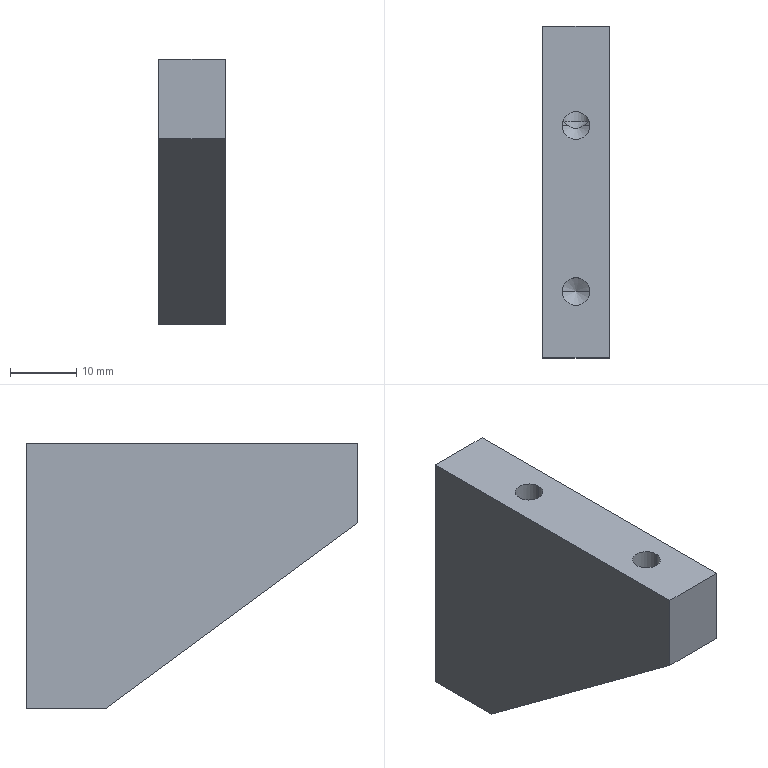Component | SolidWorks | LD101-02--Q1000-Q16-1.SLDQ1SM-1_LD101-02--Q1110-1-2 | 1 solid | 25 faces | box 10 x 50 x 40 mm | volume 13869 mm3 | cone 10 | cylinder 8 | plane 7 | commonest cylinder face diameters 4.2 x8 | material AL6061
build123d program:
from build123d import *

# Parameters (mm, degrees)
BOSS_EXTRUDE1_DEPTH   = 5
M5_TAPPED_HOLE1_D     = 4.2
M5_TAPPED_HOLE1_DEPTH = 14.4
M5_TAPPED_HOLE1_TIP   = 1.262
M5_TAPPED_HOLE2_D     = 4.2
M5_TAPPED_HOLE2_DEPTH = 14.4
M5_TAPPED_HOLE2_TIP   = 1.262


with BuildPart() as part:
    # Sketch1 → Boss-Extrude1 (new, symmetric)
    with BuildSketch(Plane.XY):
        Polygon((0, 0), (40, 0), (40, 12), (12, 50), (0, 50), align=None)
    extrude(amount=BOSS_EXTRUDE1_DEPTH, both=True)

    # M5 Tapped Hole1
    with Locations(Plane(origin=(0, 0, 0), x_dir=(-1, 0, 0), z_dir=(0, -1, 0))):
        with Locations((-15, 0), (-30, 0)):
            Hole(M5_TAPPED_HOLE1_D / 2, depth=M5_TAPPED_HOLE1_DEPTH)
            with Locations((0, 0, -(M5_TAPPED_HOLE1_DEPTH + M5_TAPPED_HOLE1_TIP / 2))):  # 118° drill point
                Cone(0, M5_TAPPED_HOLE1_D / 2, M5_TAPPED_HOLE1_TIP, mode=Mode.SUBTRACT)

    # M5 Tapped Hole2
    with Locations(Plane.ZY):
        with Locations((0, 15), (0, 40)):
            Hole(M5_TAPPED_HOLE2_D / 2, depth=M5_TAPPED_HOLE2_DEPTH)
            with Locations((0, 0, -(M5_TAPPED_HOLE2_DEPTH + M5_TAPPED_HOLE2_TIP / 2))):  # 118° drill point
                Cone(0, M5_TAPPED_HOLE2_D / 2, M5_TAPPED_HOLE2_TIP, mode=Mode.SUBTRACT)


solid = part.part

# Placed as in the assembly
solid = solid.moved(Location((-735.29, -139.897, -12.743), (180, -90, 0)))
STEP:
#1=CARTESIAN_POINT('',(-28.905,-6.098,-1.092));
#2=VERTEX_POINT('',#1);
#3=CARTESIAN_POINT('',(-28.869,-6.075,-1.069));
#4=VERTEX_POINT('',#3);
#5=CARTESIAN_POINT('',(-28.905,-6.098,-1.092));
#6=CARTESIAN_POINT('',(-28.893,-6.091,-1.085));
#7=CARTESIAN_POINT('',(-28.881,-6.083,-1.077));
#8=CARTESIAN_POINT('',(-28.869,-6.075,-1.069));
#9=B_SPLINE_CURVE_WITH_KNOTS('',3,(#5,#6,#7,#8),.UNSPECIFIED.,.F.,.F.,(4,4),(0.003787,0.005033),.UNSPECIFIED.);
#10=EDGE_CURVE('',#2,#4,#9,.T.);
#11=ORIENTED_EDGE('',*,*,#10,.F.);
#12=CARTESIAN_POINT('',(-28.866,-6.098,-1.069));
#13=VERTEX_POINT('',#12);
#14=CARTESIAN_POINT('',(-28.866,-6.098,-1.069));
#15=DIRECTION('',(0.8572,-0.,0.515));
#16=VECTOR('',#15,39.37);
#17=LINE('',#14,#16);
#18=EDGE_CURVE('',#2,#13,#17,.T.);
#19=ORIENTED_EDGE('',*,*,#18,.T.);
#20=CARTESIAN_POINT('',(-28.948,-6.098,-1.069));
#21=DIRECTION('',(-0.,-0.,1.));
#22=DIRECTION('',(-1.,0.,0.));
#23=AXIS2_PLACEMENT_3D('',#20,#21,#22);
#24=CIRCLE('',#23,0.08268);
#25=EDGE_CURVE('',#13,#4,#24,.T.);
#26=ORIENTED_EDGE('',*,*,#25,.T.);
#27=EDGE_LOOP('',(#11,#19,#26));
#28=FACE_OUTER_BOUND('',#27,.T.);
#29=CARTESIAN_POINT('',(-28.948,-6.098,-1.069));
#30=DIRECTION('',(-0.,-0.,1.));
#31=DIRECTION('',(-1.,0.,0.));
#32=AXIS2_PLACEMENT_3D('',#29,#30,#31);
#33=CONICAL_SURFACE('',#32,0.08268,1.03);
#34=ADVANCED_FACE('',(#28),#33,.F.);
#35=ORIENTED_EDGE('',*,*,#18,.F.);
#36=CARTESIAN_POINT('',(-28.992,-6.098,-1.092));
#37=VERTEX_POINT('',#36);
#38=CARTESIAN_POINT('',(-28.992,-6.098,-1.092));
#39=CARTESIAN_POINT('',(-28.985,-6.102,-1.096));
#40=CARTESIAN_POINT('',(-28.979,-6.106,-1.1));
#41=CARTESIAN_POINT('',(-28.968,-6.11,-1.104));
#42=CARTESIAN_POINT('',(-28.965,-6.112,-1.106));
#43=CARTESIAN_POINT('',(-28.957,-6.114,-1.108));
#44=CARTESIAN_POINT('',(-28.953,-6.115,-1.109));
#45=CARTESIAN_POINT('',(-28.944,-6.115,-1.109));
#46=CARTESIAN_POINT('',(-28.94,-6.114,-1.108));
#47=CARTESIAN_POINT('',(-28.932,-6.112,-1.106));
#48=CARTESIAN_POINT('',(-28.929,-6.11,-1.104));
#49=CARTESIAN_POINT('',(-28.918,-6.106,-1.1));
#50=CARTESIAN_POINT('',(-28.911,-6.102,-1.096));
#51=CARTESIAN_POINT('',(-28.905,-6.098,-1.092));
#52=B_SPLINE_CURVE_WITH_KNOTS('',3,(#38,#39,#40,#41,#42,#43,#44,#45,#46,#47,#48,#49,#50,#51),.UNSPECIFIED.,.F.,.F.,(4,2,2,2,2,2,4),(0.001245,0.001881,0.002198,0.002516,0.002834,0.003151,0.003787),.UNSPECIFIED.);
#53=EDGE_CURVE('',#37,#2,#52,.T.);
#54=ORIENTED_EDGE('',*,*,#53,.F.);
#55=CARTESIAN_POINT('',(-29.031,-6.098,-1.069));
#56=VERTEX_POINT('',#55);
#57=CARTESIAN_POINT('',(-29.031,-6.098,-1.069));
#58=DIRECTION('',(-0.8572,-0.,0.515));
#59=VECTOR('',#58,39.37);
#60=LINE('',#57,#59);
#61=EDGE_CURVE('',#37,#56,#60,.T.);
#62=ORIENTED_EDGE('',*,*,#61,.T.);
#63=CARTESIAN_POINT('',(-28.948,-6.098,-1.069));
#64=DIRECTION('',(-0.,-0.,1.));
#65=DIRECTION('',(-1.,0.,0.));
#66=AXIS2_PLACEMENT_3D('',#63,#64,#65);
#67=CIRCLE('',#66,0.08268);
#68=EDGE_CURVE('',#56,#13,#67,.T.);
#69=ORIENTED_EDGE('',*,*,#68,.T.);
#70=EDGE_LOOP('',(#35,#54,#62,#69));
#71=FACE_OUTER_BOUND('',#70,.T.);
#72=CARTESIAN_POINT('',(-28.948,-6.098,-1.069));
#73=DIRECTION('',(-0.,-0.,1.));
#74=DIRECTION('',(-1.,0.,0.));
#75=AXIS2_PLACEMENT_3D('',#72,#73,#74);
#76=CONICAL_SURFACE('',#75,0.08268,1.03);
#77=ADVANCED_FACE('',(#71),#76,.F.);
#78=ORIENTED_EDGE('',*,*,#25,.F.);
#79=CARTESIAN_POINT('',(-28.866,-6.098,-0.5017));
#80=VERTEX_POINT('',#79);
#81=CARTESIAN_POINT('',(-28.866,-6.098,-0.5017));
#82=DIRECTION('',(-0.,-0.,1.));
#83=VECTOR('',#82,39.37);
#84=LINE('',#81,#83);
#85=EDGE_CURVE('',#13,#80,#84,.T.);
#86=ORIENTED_EDGE('',*,*,#85,.T.);
#87=CARTESIAN_POINT('',(-29.031,-6.098,-0.5017));
#88=VERTEX_POINT('',#87);
#89=CARTESIAN_POINT('',(-28.948,-6.098,-0.5017));
#90=DIRECTION('',(-0.,-0.,1.));
#91=DIRECTION('',(-1.,0.,0.));
#92=AXIS2_PLACEMENT_3D('',#89,#90,#91);
#93=CIRCLE('',#92,0.08268);
#94=EDGE_CURVE('',#80,#88,#93,.T.);
#95=ORIENTED_EDGE('',*,*,#94,.T.);
#96=CARTESIAN_POINT('',(-29.031,-6.098,-0.5017));
#97=DIRECTION('',(-0.,-0.,1.));
#98=VECTOR('',#97,39.37);
#99=LINE('',#96,#98);
#100=EDGE_CURVE('',#56,#88,#99,.T.);
#101=ORIENTED_EDGE('',*,*,#100,.F.);
#102=CARTESIAN_POINT('',(-29.028,-6.075,-1.069));
#103=VERTEX_POINT('',#102);
#104=CARTESIAN_POINT('',(-28.948,-6.098,-1.069));
#105=DIRECTION('',(-0.,-0.,1.));
#106=DIRECTION('',(-1.,0.,0.));
#107=AXIS2_PLACEMENT_3D('',#104,#105,#106);
#108=CIRCLE('',#107,0.08268);
#109=EDGE_CURVE('',#103,#56,#108,.T.);
#110=ORIENTED_EDGE('',*,*,#109,.F.);
#111=CARTESIAN_POINT('',(-28.869,-6.075,-1.069));
#112=CARTESIAN_POINT('',(-28.898,-5.978,-0.972));
#113=CARTESIAN_POINT('',(-28.999,-5.978,-0.972));
#114=CARTESIAN_POINT('',(-29.028,-6.075,-1.069));
#115=(BOUNDED_CURVE()B_SPLINE_CURVE(3,(#111,#112,#113,#114),.UNSPECIFIED.,.F.,.T.)B_SPLINE_CURVE_WITH_KNOTS((4,4),(5.002,7.564),.UNSPECIFIED.)CURVE()GEOMETRIC_REPRESENTATION_ITEM()RATIONAL_B_SPLINE_CURVE((1.,0.5238,0.5238,1.))REPRESENTATION_ITEM(''));
#116=EDGE_CURVE('',#4,#103,#115,.T.);
#117=ORIENTED_EDGE('',*,*,#116,.F.);
#118=EDGE_LOOP('',(#78,#86,#95,#101,#110,#117));
#119=FACE_OUTER_BOUND('',#118,.T.);
#120=CARTESIAN_POINT('',(-28.948,-6.098,-0.5017));
#121=DIRECTION('',(-0.,-0.,1.));
#122=DIRECTION('',(-1.,0.,0.));
#123=AXIS2_PLACEMENT_3D('',#120,#121,#122);
#124=CYLINDRICAL_SURFACE('',#123,0.08268);
#125=ADVANCED_FACE('',(#119),#124,.F.);
#126=CARTESIAN_POINT('',(-28.866,-7.083,-1.069));
#127=VERTEX_POINT('',#126);
#128=CARTESIAN_POINT('',(-29.031,-7.083,-1.069));
#129=VERTEX_POINT('',#128);
#130=CARTESIAN_POINT('',(-28.948,-7.083,-1.069));
#131=DIRECTION('',(-0.,-0.,1.));
#132=DIRECTION('',(-1.,0.,0.));
#133=AXIS2_PLACEMENT_3D('',#130,#131,#132);
#134=CIRCLE('',#133,0.08268);
#135=EDGE_CURVE('',#127,#129,#134,.T.);
#136=ORIENTED_EDGE('',*,*,#135,.F.);
#137=CARTESIAN_POINT('',(-28.866,-7.083,-0.5017));
#138=VERTEX_POINT('',#137);
#139=CARTESIAN_POINT('',(-28.866,-7.083,-0.5017));
#140=DIRECTION('',(-0.,-0.,1.));
#141=VECTOR('',#140,39.37);
#142=LINE('',#139,#141);
#143=EDGE_CURVE('',#127,#138,#142,.T.);
#144=ORIENTED_EDGE('',*,*,#143,.T.);
#145=CARTESIAN_POINT('',(-29.031,-7.083,-0.5017));
#146=VERTEX_POINT('',#145);
#147=CARTESIAN_POINT('',(-28.948,-7.083,-0.5017));
#148=DIRECTION('',(-0.,-0.,1.));
#149=DIRECTION('',(-1.,0.,0.));
#150=AXIS2_PLACEMENT_3D('',#147,#148,#149);
#151=CIRCLE('',#150,0.08268);
#152=EDGE_CURVE('',#138,#146,#151,.T.);
#153=ORIENTED_EDGE('',*,*,#152,.T.);
#154=CARTESIAN_POINT('',(-29.031,-7.083,-0.5017));
#155=DIRECTION('',(-0.,-0.,1.));
#156=VECTOR('',#155,39.37);
#157=LINE('',#154,#156);
#158=EDGE_CURVE('',#129,#146,#157,.T.);
#159=ORIENTED_EDGE('',*,*,#158,.F.);
#160=EDGE_LOOP('',(#136,#144,#153,#159));
#161=FACE_OUTER_BOUND('',#160,.T.);
#162=CARTESIAN_POINT('',(-28.948,-7.083,-0.5017));
#163=DIRECTION('',(-0.,-0.,1.));
#164=DIRECTION('',(-1.,0.,0.));
#165=AXIS2_PLACEMENT_3D('',#162,#163,#164);
#166=CYLINDRICAL_SURFACE('',#165,0.08268);
#167=ADVANCED_FACE('',(#161),#166,.F.);
#168=CARTESIAN_POINT('',(-28.948,-7.083,-1.118));
#169=VERTEX_POINT('',#168);
#170=CARTESIAN_POINT('',(-29.031,-7.083,-1.069));
#171=DIRECTION('',(-0.8572,-0.,0.515));
#172=VECTOR('',#171,39.37);
#173=LINE('',#170,#172);
#174=EDGE_CURVE('',#169,#129,#173,.T.);
#175=ORIENTED_EDGE('',*,*,#174,.F.);
#176=CARTESIAN_POINT('',(-28.866,-7.083,-1.069));
#177=DIRECTION('',(0.8572,-0.,0.515));
#178=VECTOR('',#177,39.37);
#179=LINE('',#176,#178);
#180=EDGE_CURVE('',#169,#127,#179,.T.);
#181=ORIENTED_EDGE('',*,*,#180,.T.);
#182=ORIENTED_EDGE('',*,*,#135,.T.);
#183=EDGE_LOOP('',(#175,#181,#182));
#184=FACE_OUTER_BOUND('',#183,.T.);
#185=CARTESIAN_POINT('',(-28.948,-7.083,-1.069));
#186=DIRECTION('',(-0.,-0.,1.));
#187=DIRECTION('',(-1.,0.,0.));
#188=AXIS2_PLACEMENT_3D('',#185,#186,#187);
#189=CONICAL_SURFACE('',#188,0.08268,1.03);
#190=ADVANCED_FACE('',(#184),#189,.F.);
#191=CARTESIAN_POINT('',(-29.031,-6.075,-1.092));
#192=VERTEX_POINT('',#191);
#193=CARTESIAN_POINT('',(-28.948,-6.075,-1.092));
#194=DIRECTION('',(0.,1.,0.));
#195=DIRECTION('',(1.,0.,0.));
#196=AXIS2_PLACEMENT_3D('',#193,#194,#195);
#197=CIRCLE('',#196,0.08268);
#198=EDGE_CURVE('',#192,#103,#197,.T.);
#199=ORIENTED_EDGE('',*,*,#198,.F.);
#200=CARTESIAN_POINT('',(-29.031,-5.508,-1.092));
#201=VERTEX_POINT('',#200);
#202=CARTESIAN_POINT('',(-29.031,-5.508,-1.092));
#203=DIRECTION('',(0.,1.,0.));
#204=VECTOR('',#203,39.37);
#205=LINE('',#202,#204);
#206=EDGE_CURVE('',#192,#201,#205,.T.);
#207=ORIENTED_EDGE('',*,*,#206,.T.);
#208=CARTESIAN_POINT('',(-28.866,-5.508,-1.092));
#209=VERTEX_POINT('',#208);
#210=CARTESIAN_POINT('',(-28.948,-5.508,-1.092));
#211=DIRECTION('',(0.,1.,0.));
#212=DIRECTION('',(1.,0.,0.));
#213=AXIS2_PLACEMENT_3D('',#210,#211,#212);
#214=CIRCLE('',#213,0.08268);
#215=EDGE_CURVE('',#201,#209,#214,.T.);
#216=ORIENTED_EDGE('',*,*,#215,.T.);
#217=CARTESIAN_POINT('',(-28.866,-6.075,-1.092));
#218=VERTEX_POINT('',#217);
#219=CARTESIAN_POINT('',(-28.866,-5.508,-1.092));
#220=DIRECTION('',(0.,1.,0.));
#221=VECTOR('',#220,39.37);
#222=LINE('',#219,#221);
#223=EDGE_CURVE('',#218,#209,#222,.T.);
#224=ORIENTED_EDGE('',*,*,#223,.F.);
#225=CARTESIAN_POINT('',(-28.948,-6.075,-1.092));
#226=DIRECTION('',(0.,1.,0.));
#227=DIRECTION('',(1.,0.,0.));
#228=AXIS2_PLACEMENT_3D('',#225,#226,#227);
#229=CIRCLE('',#228,0.08268);
#230=EDGE_CURVE('',#4,#218,#229,.T.);
#231=ORIENTED_EDGE('',*,*,#230,.F.);
#232=ORIENTED_EDGE('',*,*,#116,.T.);
#233=EDGE_LOOP('',(#199,#207,#216,#224,#231,#232));
#234=FACE_OUTER_BOUND('',#233,.T.);
#235=CARTESIAN_POINT('',(-28.948,-5.508,-1.092));
#236=DIRECTION('',(0.,1.,0.));
#237=DIRECTION('',(1.,0.,0.));
#238=AXIS2_PLACEMENT_3D('',#235,#236,#237);
#239=CYLINDRICAL_SURFACE('',#238,0.08268);
#240=ADVANCED_FACE('',(#234),#239,.F.);
#241=CARTESIAN_POINT('',(-29.028,-6.075,-1.069));
#242=CARTESIAN_POINT('',(-29.016,-6.083,-1.077));
#243=CARTESIAN_POINT('',(-29.004,-6.091,-1.085));
#244=CARTESIAN_POINT('',(-28.992,-6.098,-1.092));
#245=B_SPLINE_CURVE_WITH_KNOTS('',3,(#241,#242,#243,#244),.UNSPECIFIED.,.F.,.F.,(4,4),(0.0000004,0.001245),.UNSPECIFIED.);
#246=EDGE_CURVE('',#103,#37,#245,.T.);
#247=ORIENTED_EDGE('',*,*,#246,.T.);
#248=CARTESIAN_POINT('',(-29.031,-6.075,-1.092));
#249=DIRECTION('',(-0.8572,0.515,-0.));
#250=VECTOR('',#249,39.37);
#251=LINE('',#248,#250);
#252=EDGE_CURVE('',#37,#192,#251,.T.);
#253=ORIENTED_EDGE('',*,*,#252,.T.);
#254=ORIENTED_EDGE('',*,*,#198,.T.);
#255=EDGE_LOOP('',(#247,#253,#254));
#256=FACE_OUTER_BOUND('',#255,.T.);
#257=CARTESIAN_POINT('',(-28.948,-6.075,-1.092));
#258=DIRECTION('',(0.,1.,0.));
#259=DIRECTION('',(1.,0.,0.));
#260=AXIS2_PLACEMENT_3D('',#257,#258,#259);
#261=CONICAL_SURFACE('',#260,0.08268,1.03);
#262=ADVANCED_FACE('',(#256),#261,.F.);
#263=ORIENTED_EDGE('',*,*,#252,.F.);
#264=ORIENTED_EDGE('',*,*,#53,.T.);
#265=CARTESIAN_POINT('',(-28.866,-6.075,-1.092));
#266=DIRECTION('',(0.8572,0.515,0.));
#267=VECTOR('',#266,39.37);
#268=LINE('',#265,#267);
#269=EDGE_CURVE('',#2,#218,#268,.T.);
#270=ORIENTED_EDGE('',*,*,#269,.T.);
#271=CARTESIAN_POINT('',(-28.948,-6.075,-1.092));
#272=DIRECTION('',(0.,1.,0.));
#273=DIRECTION('',(1.,0.,0.));
#274=AXIS2_PLACEMENT_3D('',#271,#272,#273);
#275=CIRCLE('',#274,0.08268);
#276=EDGE_CURVE('',#218,#192,#275,.T.);
#277=ORIENTED_EDGE('',*,*,#276,.T.);
#278=EDGE_LOOP('',(#263,#264,#270,#277));
#279=FACE_OUTER_BOUND('',#278,.T.);
#280=CARTESIAN_POINT('',(-28.948,-6.075,-1.092));
#281=DIRECTION('',(0.,1.,0.));
#282=DIRECTION('',(1.,0.,0.));
#283=AXIS2_PLACEMENT_3D('',#280,#281,#282);
#284=CONICAL_SURFACE('',#283,0.08268,1.03);
#285=ADVANCED_FACE('',(#279),#284,.F.);
#286=CARTESIAN_POINT('',(-29.031,-6.075,-1.683));
#287=VERTEX_POINT('',#286);
#288=CARTESIAN_POINT('',(-28.866,-6.075,-1.683));
#289=VERTEX_POINT('',#288);
#290=CARTESIAN_POINT('',(-28.948,-6.075,-1.683));
#291=DIRECTION('',(0.,1.,0.));
#292=DIRECTION('',(1.,0.,0.));
#293=AXIS2_PLACEMENT_3D('',#290,#291,#292);
#294=CIRCLE('',#293,0.08268);
#295=EDGE_CURVE('',#287,#289,#294,.T.);
#296=ORIENTED_EDGE('',*,*,#295,.F.);
#297=CARTESIAN_POINT('',(-29.031,-5.508,-1.683));
#298=VERTEX_POINT('',#297);
#299=CARTESIAN_POINT('',(-29.031,-5.508,-1.683));
#300=DIRECTION('',(0.,1.,0.));
#301=VECTOR('',#300,39.37);
#302=LINE('',#299,#301);
#303=EDGE_CURVE('',#287,#298,#302,.T.);
#304=ORIENTED_EDGE('',*,*,#303,.T.);
#305=CARTESIAN_POINT('',(-28.866,-5.508,-1.683));
#306=VERTEX_POINT('',#305);
#307=CARTESIAN_POINT('',(-28.948,-5.508,-1.683));
#308=DIRECTION('',(0.,1.,0.));
#309=DIRECTION('',(1.,0.,0.));
#310=AXIS2_PLACEMENT_3D('',#307,#308,#309);
#311=CIRCLE('',#310,0.08268);
#312=EDGE_CURVE('',#298,#306,#311,.T.);
#313=ORIENTED_EDGE('',*,*,#312,.T.);
#314=CARTESIAN_POINT('',(-28.866,-5.508,-1.683));
#315=DIRECTION('',(0.,1.,0.));
#316=VECTOR('',#315,39.37);
#317=LINE('',#314,#316);
#318=EDGE_CURVE('',#289,#306,#317,.T.);
#319=ORIENTED_EDGE('',*,*,#318,.F.);
#320=EDGE_LOOP('',(#296,#304,#313,#319));
#321=FACE_OUTER_BOUND('',#320,.T.);
#322=CARTESIAN_POINT('',(-28.948,-5.508,-1.683));
#323=DIRECTION('',(0.,1.,0.));
#324=DIRECTION('',(1.,0.,0.));
#325=AXIS2_PLACEMENT_3D('',#322,#323,#324);
#326=CYLINDRICAL_SURFACE('',#325,0.08268);
#327=ADVANCED_FACE('',(#321),#326,.F.);
#328=CARTESIAN_POINT('',(-28.948,-6.124,-1.683));
#329=VERTEX_POINT('',#328);
#330=CARTESIAN_POINT('',(-28.866,-6.075,-1.683));
#331=DIRECTION('',(0.8572,0.515,0.));
#332=VECTOR('',#331,39.37);
#333=LINE('',#330,#332);
#334=EDGE_CURVE('',#329,#289,#333,.T.);
#335=ORIENTED_EDGE('',*,*,#334,.F.);
#336=CARTESIAN_POINT('',(-29.031,-6.075,-1.683));
#337=DIRECTION('',(-0.8572,0.515,-0.));
#338=VECTOR('',#337,39.37);
#339=LINE('',#336,#338);
#340=EDGE_CURVE('',#329,#287,#339,.T.);
#341=ORIENTED_EDGE('',*,*,#340,.T.);
#342=ORIENTED_EDGE('',*,*,#295,.T.);
#343=EDGE_LOOP('',(#335,#341,#342));
#344=FACE_OUTER_BOUND('',#343,.T.);
#345=CARTESIAN_POINT('',(-28.948,-6.075,-1.683));
#346=DIRECTION('',(0.,1.,0.));
#347=DIRECTION('',(1.,0.,0.));
#348=AXIS2_PLACEMENT_3D('',#345,#346,#347);
#349=CONICAL_SURFACE('',#348,0.08268,1.03);
#350=ADVANCED_FACE('',(#344),#349,.F.);
#351=CARTESIAN_POINT('',(-28.948,-6.098,-0.5017));
#352=DIRECTION('',(-0.,-0.,1.));
#353=DIRECTION('',(-1.,0.,0.));
#354=AXIS2_PLACEMENT_3D('',#351,#352,#353);
#355=CIRCLE('',#354,0.08268);
#356=EDGE_CURVE('',#88,#80,#355,.T.);
#357=ORIENTED_EDGE('',*,*,#356,.F.);
#358=ORIENTED_EDGE('',*,*,#94,.F.);
#359=EDGE_LOOP('',(#357,#358));
#360=FACE_BOUND('',#359,.T.);
#361=CARTESIAN_POINT('',(-28.948,-7.083,-0.5017));
#362=DIRECTION('',(-0.,-0.,1.));
#363=DIRECTION('',(-1.,0.,0.));
#364=AXIS2_PLACEMENT_3D('',#361,#362,#363);
#365=CIRCLE('',#364,0.08268);
#366=EDGE_CURVE('',#146,#138,#365,.T.);
#367=ORIENTED_EDGE('',*,*,#366,.F.);
#368=ORIENTED_EDGE('',*,*,#152,.F.);
#369=EDGE_LOOP('',(#367,#368));
#370=FACE_BOUND('',#369,.T.);
#371=CARTESIAN_POINT('',(-28.752,-7.476,-0.5017));
#372=VERTEX_POINT('',#371);
#373=CARTESIAN_POINT('',(-28.752,-5.508,-0.5017));
#374=VERTEX_POINT('',#373);
#375=CARTESIAN_POINT('',(-28.752,-7.476,-0.5017));
#376=DIRECTION('',(0.,1.,-0.));
#377=VECTOR('',#376,39.37);
#378=LINE('',#375,#377);
#379=EDGE_CURVE('',#372,#374,#378,.T.);
#380=ORIENTED_EDGE('',*,*,#379,.T.);
#381=CARTESIAN_POINT('',(-29.145,-5.508,-0.5017));
#382=VERTEX_POINT('',#381);
#383=CARTESIAN_POINT('',(-29.145,-5.508,-0.5017));
#384=DIRECTION('',(1.,-0.,0.));
#385=VECTOR('',#384,39.37);
#386=LINE('',#383,#385);
#387=EDGE_CURVE('',#382,#374,#386,.T.);
#388=ORIENTED_EDGE('',*,*,#387,.F.);
#389=CARTESIAN_POINT('',(-29.145,-7.476,-0.5017));
#390=VERTEX_POINT('',#389);
#391=CARTESIAN_POINT('',(-29.145,-7.476,-0.5017));
#392=DIRECTION('',(0.,1.,-0.));
#393=VECTOR('',#392,39.37);
#394=LINE('',#391,#393);
#395=EDGE_CURVE('',#390,#382,#394,.T.);
#396=ORIENTED_EDGE('',*,*,#395,.F.);
#397=CARTESIAN_POINT('',(-29.145,-7.476,-0.5017));
#398=DIRECTION('',(1.,-0.,0.));
#399=VECTOR('',#398,39.37);
#400=LINE('',#397,#399);
#401=EDGE_CURVE('',#390,#372,#400,.T.);
#402=ORIENTED_EDGE('',*,*,#401,.T.);
#403=EDGE_LOOP('',(#380,#388,#396,#402));
#404=FACE_OUTER_BOUND('',#403,.T.);
#405=CARTESIAN_POINT('',(-29.145,-7.476,-0.5017));
#406=DIRECTION('',(0.,-0.,-1.));
#407=DIRECTION('',(-0.,-1.,0.));
#408=AXIS2_PLACEMENT_3D('',#405,#406,#407);
#409=PLANE('',#408);
#410=ADVANCED_FACE('',(#360,#370,#404),#409,.F.);
#411=CARTESIAN_POINT('',(-28.948,-5.508,-1.092));
#412=DIRECTION('',(0.,1.,0.));
#413=DIRECTION('',(1.,0.,0.));
#414=AXIS2_PLACEMENT_3D('',#411,#412,#413);
#415=CIRCLE('',#414,0.08268);
#416=EDGE_CURVE('',#209,#201,#415,.T.);
#417=ORIENTED_EDGE('',*,*,#416,.F.);
#418=ORIENTED_EDGE('',*,*,#215,.F.);
#419=EDGE_LOOP('',(#417,#418));
#420=FACE_BOUND('',#419,.T.);
#421=CARTESIAN_POINT('',(-28.948,-5.508,-1.683));
#422=DIRECTION('',(0.,1.,0.));
#423=DIRECTION('',(1.,0.,0.));
#424=AXIS2_PLACEMENT_3D('',#421,#422,#423);
#425=CIRCLE('',#424,0.08268);
#426=EDGE_CURVE('',#306,#298,#425,.T.);
#427=ORIENTED_EDGE('',*,*,#426,.F.);
#428=ORIENTED_EDGE('',*,*,#312,.F.);
#429=EDGE_LOOP('',(#427,#428));
#430=FACE_BOUND('',#429,.T.);
#431=CARTESIAN_POINT('',(-28.752,-5.508,-2.077));
#432=VERTEX_POINT('',#431);
#433=CARTESIAN_POINT('',(-28.752,-5.508,-0.5017));
#434=DIRECTION('',(0.,0.,-1.));
#435=VECTOR('',#434,39.37);
#436=LINE('',#433,#435);
#437=EDGE_CURVE('',#374,#432,#436,.T.);
#438=ORIENTED_EDGE('',*,*,#437,.T.);
#439=CARTESIAN_POINT('',(-29.145,-5.508,-2.077));
#440=VERTEX_POINT('',#439);
#441=CARTESIAN_POINT('',(-29.145,-5.508,-2.077));
#442=DIRECTION('',(1.,-0.,0.));
#443=VECTOR('',#442,39.37);
#444=LINE('',#441,#443);
#445=EDGE_CURVE('',#440,#432,#444,.T.);
#446=ORIENTED_EDGE('',*,*,#445,.F.);
#447=CARTESIAN_POINT('',(-29.145,-5.508,-0.5017));
#448=DIRECTION('',(0.,0.,-1.));
#449=VECTOR('',#448,39.37);
#450=LINE('',#447,#449);
#451=EDGE_CURVE('',#382,#440,#450,.T.);
#452=ORIENTED_EDGE('',*,*,#451,.F.);
#453=ORIENTED_EDGE('',*,*,#387,.T.);
#454=EDGE_LOOP('',(#438,#446,#452,#453));
#455=FACE_OUTER_BOUND('',#454,.T.);
#456=CARTESIAN_POINT('',(-29.145,-5.508,-0.5017));
#457=DIRECTION('',(-0.,-1.,-0.));
#458=DIRECTION('',(-1.,0.,-0.));
#459=AXIS2_PLACEMENT_3D('',#456,#457,#458);
#460=PLANE('',#459);
#461=ADVANCED_FACE('',(#420,#430,#455),#460,.F.);
#462=CARTESIAN_POINT('',(-28.752,-5.98,-2.077));
#463=VERTEX_POINT('',#462);
#464=CARTESIAN_POINT('',(-28.752,-5.508,-2.077));
#465=DIRECTION('',(-0.,-1.,-0.));
#466=VECTOR('',#465,39.37);
#467=LINE('',#464,#466);
#468=EDGE_CURVE('',#432,#463,#467,.T.);
#469=ORIENTED_EDGE('',*,*,#468,.T.);
#470=CARTESIAN_POINT('',(-29.145,-5.98,-2.077));
#471=VERTEX_POINT('',#470);
#472=CARTESIAN_POINT('',(-29.145,-5.98,-2.077));
#473=DIRECTION('',(1.,-0.,0.));
#474=VECTOR('',#473,39.37);
#475=LINE('',#472,#474);
#476=EDGE_CURVE('',#471,#463,#475,.T.);
#477=ORIENTED_EDGE('',*,*,#476,.F.);
#478=CARTESIAN_POINT('',(-29.145,-5.508,-2.077));
#479=DIRECTION('',(-0.,-1.,-0.));
#480=VECTOR('',#479,39.37);
#481=LINE('',#478,#480);
#482=EDGE_CURVE('',#440,#471,#481,.T.);
#483=ORIENTED_EDGE('',*,*,#482,.F.);
#484=ORIENTED_EDGE('',*,*,#445,.T.);
#485=EDGE_LOOP('',(#469,#477,#483,#484));
#486=FACE_OUTER_BOUND('',#485,.T.);
#487=CARTESIAN_POINT('',(-29.145,-5.508,-2.077));
#488=DIRECTION('',(-0.,-0.,1.));
#489=DIRECTION('',(-1.,0.,-0.));
#490=AXIS2_PLACEMENT_3D('',#487,#488,#489);
#491=PLANE('',#490);
#492=ADVANCED_FACE('',(#486),#491,.F.);
#493=CARTESIAN_POINT('',(-28.752,-7.476,-0.9741));
#494=VERTEX_POINT('',#493);
#495=CARTESIAN_POINT('',(-28.752,-5.98,-2.077));
#496=DIRECTION('',(-0.,-0.8051,0.5932));
#497=VECTOR('',#496,39.37);
#498=LINE('',#495,#497);
#499=EDGE_CURVE('',#463,#494,#498,.T.);
#500=ORIENTED_EDGE('',*,*,#499,.T.);
#501=CARTESIAN_POINT('',(-29.145,-7.476,-0.9741));
#502=VERTEX_POINT('',#501);
#503=CARTESIAN_POINT('',(-29.145,-7.476,-0.9741));
#504=DIRECTION('',(1.,-0.,0.));
#505=VECTOR('',#504,39.37);
#506=LINE('',#503,#505);
#507=EDGE_CURVE('',#502,#494,#506,.T.);
#508=ORIENTED_EDGE('',*,*,#507,.F.);
#509=CARTESIAN_POINT('',(-29.145,-5.98,-2.077));
#510=DIRECTION('',(-0.,-0.8051,0.5932));
#511=VECTOR('',#510,39.37);
#512=LINE('',#509,#511);
#513=EDGE_CURVE('',#471,#502,#512,.T.);
#514=ORIENTED_EDGE('',*,*,#513,.F.);
#515=ORIENTED_EDGE('',*,*,#476,.T.);
#516=EDGE_LOOP('',(#500,#508,#514,#515));
#517=FACE_OUTER_BOUND('',#516,.T.);
#518=CARTESIAN_POINT('',(-29.145,-5.98,-2.077));
#519=DIRECTION('',(-0.,0.5932,0.8051));
#520=DIRECTION('',(0.,0.8051,-0.5932));
#521=AXIS2_PLACEMENT_3D('',#518,#519,#520);
#522=PLANE('',#521);
#523=ADVANCED_FACE('',(#517),#522,.F.);
#524=CARTESIAN_POINT('',(-28.752,-7.476,-0.9741));
#525=DIRECTION('',(-0.,-0.,1.));
#526=VECTOR('',#525,39.37);
#527=LINE('',#524,#526);
#528=EDGE_CURVE('',#494,#372,#527,.T.);
#529=ORIENTED_EDGE('',*,*,#528,.T.);
#530=ORIENTED_EDGE('',*,*,#401,.F.);
#531=CARTESIAN_POINT('',(-29.145,-7.476,-0.9741));
#532=DIRECTION('',(-0.,-0.,1.));
#533=VECTOR('',#532,39.37);
#534=LINE('',#531,#533);
#535=EDGE_CURVE('',#502,#390,#534,.T.);
#536=ORIENTED_EDGE('',*,*,#535,.F.);
#537=ORIENTED_EDGE('',*,*,#507,.T.);
#538=EDGE_LOOP('',(#529,#530,#536,#537));
#539=FACE_OUTER_BOUND('',#538,.T.);
#540=CARTESIAN_POINT('',(-29.145,-7.476,-0.9741));
#541=DIRECTION('',(0.,1.,0.));
#542=DIRECTION('',(1.,-0.,0.));
#543=AXIS2_PLACEMENT_3D('',#540,#541,#542);
#544=PLANE('',#543);
#545=ADVANCED_FACE('',(#539),#544,.F.);
#546=ORIENTED_EDGE('',*,*,#395,.T.);
#547=ORIENTED_EDGE('',*,*,#451,.T.);
#548=ORIENTED_EDGE('',*,*,#482,.T.);
#549=ORIENTED_EDGE('',*,*,#513,.T.);
#550=ORIENTED_EDGE('',*,*,#535,.T.);
#551=EDGE_LOOP('',(#546,#547,#548,#549,#550));
#552=FACE_OUTER_BOUND('',#551,.T.);
#553=CARTESIAN_POINT('',(-29.145,-5.508,-0.5017));
#554=DIRECTION('',(-1.,0.,-0.));
#555=DIRECTION('',(0.,0.,-1.));
#556=AXIS2_PLACEMENT_3D('',#553,#554,#555);
#557=PLANE('',#556);
#558=ADVANCED_FACE('',(#552),#557,.T.);
#559=ORIENTED_EDGE('',*,*,#379,.F.);
#560=ORIENTED_EDGE('',*,*,#528,.F.);
#561=ORIENTED_EDGE('',*,*,#499,.F.);
#562=ORIENTED_EDGE('',*,*,#468,.F.);
#563=ORIENTED_EDGE('',*,*,#437,.F.);
#564=EDGE_LOOP('',(#559,#560,#561,#562,#563));
#565=FACE_OUTER_BOUND('',#564,.T.);
#566=CARTESIAN_POINT('',(-28.752,-5.508,-0.5017));
#567=DIRECTION('',(-1.,0.,-0.));
#568=DIRECTION('',(0.,0.,-1.));
#569=AXIS2_PLACEMENT_3D('',#566,#567,#568);
#570=PLANE('',#569);
#571=ADVANCED_FACE('',(#565),#570,.F.);
#572=ORIENTED_EDGE('',*,*,#340,.F.);
#573=ORIENTED_EDGE('',*,*,#334,.T.);
#574=CARTESIAN_POINT('',(-28.948,-6.075,-1.683));
#575=DIRECTION('',(0.,1.,0.));
#576=DIRECTION('',(1.,0.,0.));
#577=AXIS2_PLACEMENT_3D('',#574,#575,#576);
#578=CIRCLE('',#577,0.08268);
#579=EDGE_CURVE('',#289,#287,#578,.T.);
#580=ORIENTED_EDGE('',*,*,#579,.T.);
#581=EDGE_LOOP('',(#572,#573,#580));
#582=FACE_OUTER_BOUND('',#581,.T.);
#583=CARTESIAN_POINT('',(-28.948,-6.075,-1.683));
#584=DIRECTION('',(0.,1.,0.));
#585=DIRECTION('',(1.,0.,0.));
#586=AXIS2_PLACEMENT_3D('',#583,#584,#585);
#587=CONICAL_SURFACE('',#586,0.08268,1.03);
#588=ADVANCED_FACE('',(#582),#587,.F.);
#589=ORIENTED_EDGE('',*,*,#303,.F.);
#590=ORIENTED_EDGE('',*,*,#579,.F.);
#591=ORIENTED_EDGE('',*,*,#318,.T.);
#592=ORIENTED_EDGE('',*,*,#426,.T.);
#593=EDGE_LOOP('',(#589,#590,#591,#592));
#594=FACE_OUTER_BOUND('',#593,.T.);
#595=CARTESIAN_POINT('',(-28.948,-5.508,-1.683));
#596=DIRECTION('',(0.,1.,0.));
#597=DIRECTION('',(1.,0.,0.));
#598=AXIS2_PLACEMENT_3D('',#595,#596,#597);
#599=CYLINDRICAL_SURFACE('',#598,0.08268);
#600=ADVANCED_FACE('',(#594),#599,.F.);
#601=ORIENTED_EDGE('',*,*,#269,.F.);
#602=ORIENTED_EDGE('',*,*,#10,.T.);
#603=ORIENTED_EDGE('',*,*,#230,.T.);
#604=EDGE_LOOP('',(#601,#602,#603));
#605=FACE_OUTER_BOUND('',#604,.T.);
#606=CARTESIAN_POINT('',(-28.948,-6.075,-1.092));
#607=DIRECTION('',(0.,1.,0.));
#608=DIRECTION('',(1.,0.,0.));
#609=AXIS2_PLACEMENT_3D('',#606,#607,#608);
#610=CONICAL_SURFACE('',#609,0.08268,1.03);
#611=ADVANCED_FACE('',(#605),#610,.F.);
#612=ORIENTED_EDGE('',*,*,#206,.F.);
#613=ORIENTED_EDGE('',*,*,#276,.F.);
#614=ORIENTED_EDGE('',*,*,#223,.T.);
#615=ORIENTED_EDGE('',*,*,#416,.T.);
#616=EDGE_LOOP('',(#612,#613,#614,#615));
#617=FACE_OUTER_BOUND('',#616,.T.);
#618=CARTESIAN_POINT('',(-28.948,-5.508,-1.092));
#619=DIRECTION('',(0.,1.,0.));
#620=DIRECTION('',(1.,0.,0.));
#621=AXIS2_PLACEMENT_3D('',#618,#619,#620);
#622=CYLINDRICAL_SURFACE('',#621,0.08268);
#623=ADVANCED_FACE('',(#617),#622,.F.);
#624=ORIENTED_EDGE('',*,*,#180,.F.);
#625=ORIENTED_EDGE('',*,*,#174,.T.);
#626=CARTESIAN_POINT('',(-28.948,-7.083,-1.069));
#627=DIRECTION('',(-0.,-0.,1.));
#628=DIRECTION('',(-1.,0.,0.));
#629=AXIS2_PLACEMENT_3D('',#626,#627,#628);
#630=CIRCLE('',#629,0.08268);
#631=EDGE_CURVE('',#129,#127,#630,.T.);
#632=ORIENTED_EDGE('',*,*,#631,.T.);
#633=EDGE_LOOP('',(#624,#625,#632));
#634=FACE_OUTER_BOUND('',#633,.T.);
#635=CARTESIAN_POINT('',(-28.948,-7.083,-1.069));
#636=DIRECTION('',(-0.,-0.,1.));
#637=DIRECTION('',(-1.,0.,0.));
#638=AXIS2_PLACEMENT_3D('',#635,#636,#637);
#639=CONICAL_SURFACE('',#638,0.08268,1.03);
#640=ADVANCED_FACE('',(#634),#639,.F.);
#641=ORIENTED_EDGE('',*,*,#143,.F.);
#642=ORIENTED_EDGE('',*,*,#631,.F.);
#643=ORIENTED_EDGE('',*,*,#158,.T.);
#644=ORIENTED_EDGE('',*,*,#366,.T.);
#645=EDGE_LOOP('',(#641,#642,#643,#644));
#646=FACE_OUTER_BOUND('',#645,.T.);
#647=CARTESIAN_POINT('',(-28.948,-7.083,-0.5017));
#648=DIRECTION('',(-0.,-0.,1.));
#649=DIRECTION('',(-1.,0.,0.));
#650=AXIS2_PLACEMENT_3D('',#647,#648,#649);
#651=CYLINDRICAL_SURFACE('',#650,0.08268);
#652=ADVANCED_FACE('',(#646),#651,.F.);
#653=ORIENTED_EDGE('',*,*,#85,.F.);
#654=ORIENTED_EDGE('',*,*,#68,.F.);
#655=ORIENTED_EDGE('',*,*,#100,.T.);
#656=ORIENTED_EDGE('',*,*,#356,.T.);
#657=EDGE_LOOP('',(#653,#654,#655,#656));
#658=FACE_OUTER_BOUND('',#657,.T.);
#659=CARTESIAN_POINT('',(-28.948,-6.098,-0.5017));
#660=DIRECTION('',(-0.,-0.,1.));
#661=DIRECTION('',(-1.,0.,0.));
#662=AXIS2_PLACEMENT_3D('',#659,#660,#661);
#663=CYLINDRICAL_SURFACE('',#662,0.08268);
#664=ADVANCED_FACE('',(#658),#663,.F.);
#665=ORIENTED_EDGE('',*,*,#61,.F.);
#666=ORIENTED_EDGE('',*,*,#246,.F.);
#667=ORIENTED_EDGE('',*,*,#109,.T.);
#668=EDGE_LOOP('',(#665,#666,#667));
#669=FACE_OUTER_BOUND('',#668,.T.);
#670=CARTESIAN_POINT('',(-28.948,-6.098,-1.069));
#671=DIRECTION('',(-0.,-0.,1.));
#672=DIRECTION('',(-1.,0.,0.));
#673=AXIS2_PLACEMENT_3D('',#670,#671,#672);
#674=CONICAL_SURFACE('',#673,0.08268,1.03);
#675=ADVANCED_FACE('',(#669),#674,.F.);
#676=CLOSED_SHELL('',(#34,#77,#125,#167,#190,#240,#262,#285,#327,#350,#410,#461,#492,#523,#545,#558,#571,#588,#600,#611,#623,#640,#652,#664,#675));
#677=MANIFOLD_SOLID_BREP('',#676);
#678=CARTESIAN_POINT('',(0.,0.,0.));
#679=DIRECTION('',(0.,0.,1.));
#680=DIRECTION('',(1.,0.,0.));
#681=AXIS2_PLACEMENT_3D('',#678,#679,#680);
#682=(LENGTH_UNIT()NAMED_UNIT(*)SI_UNIT($,.METRE.));
#683=LENGTH_MEASURE_WITH_UNIT(LENGTH_MEASURE(0.0254),#682);
#684=DIMENSIONAL_EXPONENTS(1.,0.,0.,0.,0.,0.,0.);
#685=(CONVERSION_BASED_UNIT('',#683)LENGTH_UNIT()NAMED_UNIT(#684));
#686=UNCERTAINTY_MEASURE_WITH_UNIT(LENGTH_MEASURE(0.00001),#685,'','');
#687=(NAMED_UNIT(*)PLANE_ANGLE_UNIT()SI_UNIT($,.RADIAN.));
#688=(NAMED_UNIT(*)SI_UNIT($,.STERADIAN.)SOLID_ANGLE_UNIT());
#689=(GEOMETRIC_REPRESENTATION_CONTEXT(3)GLOBAL_UNCERTAINTY_ASSIGNED_CONTEXT((#686))GLOBAL_UNIT_ASSIGNED_CONTEXT((#685,#687,#688))REPRESENTATION_CONTEXT('',''));
#690=ADVANCED_BREP_SHAPE_REPRESENTATION('',(#677,#681),#689);
#691=COLOUR_RGB('',0.7922,0.8196,0.9333);
#692=FILL_AREA_STYLE_COLOUR('',#691);
#693=FILL_AREA_STYLE('',(#692));
#694=SURFACE_STYLE_FILL_AREA(#693);
#695=SURFACE_SIDE_STYLE('',(#694));
#696=SURFACE_STYLE_USAGE(.BOTH.,#695);
#697=PRESENTATION_STYLE_ASSIGNMENT((#696));
#698=STYLED_ITEM('',(#697),#677);
#699=(LENGTH_UNIT()NAMED_UNIT(*)SI_UNIT($,.METRE.));
#700=LENGTH_MEASURE_WITH_UNIT(LENGTH_MEASURE(0.0254),#699);
#701=DIMENSIONAL_EXPONENTS(1.,0.,0.,0.,0.,0.,0.);
#702=(CONVERSION_BASED_UNIT('',#700)LENGTH_UNIT()NAMED_UNIT(#701));
#703=UNCERTAINTY_MEASURE_WITH_UNIT(LENGTH_MEASURE(0.00001),#702,'','');
#704=(NAMED_UNIT(*)PLANE_ANGLE_UNIT()SI_UNIT($,.RADIAN.));
#705=(NAMED_UNIT(*)SI_UNIT($,.STERADIAN.)SOLID_ANGLE_UNIT());
#706=(GEOMETRIC_REPRESENTATION_CONTEXT(3)GLOBAL_UNCERTAINTY_ASSIGNED_CONTEXT((#703))GLOBAL_UNIT_ASSIGNED_CONTEXT((#702,#704,#705))REPRESENTATION_CONTEXT('',''));
#707=MECHANICAL_DESIGN_GEOMETRIC_PRESENTATION_REPRESENTATION('',(#698),#706);
#708=PRESENTATION_LAYER_ASSIGNMENT('','',(#698));